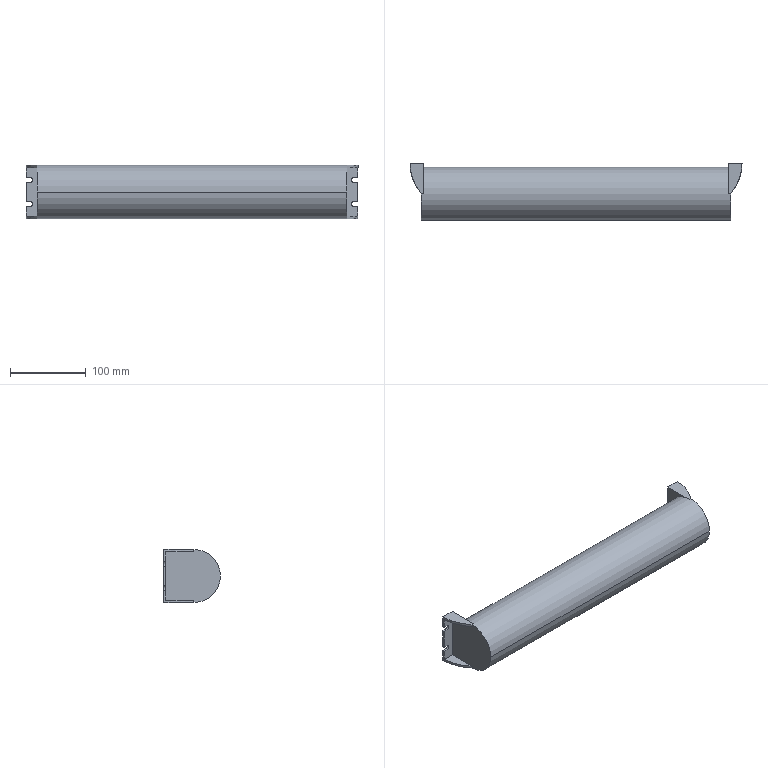Component | SolidWorks | IlluminationLamp-1 | 1 solid | 36 faces | box 438 x 75 x 70 mm | volume 1585479 mm3 | plane 24 | cylinder 12 | commonest cylinder face diameters 121.667 x6 6.5 x4 70 x2
STEP:
#1=COLOUR_RGB('',0.7922,0.8196,0.9333);
#2=FILL_AREA_STYLE_COLOUR('',#1);
#3=FILL_AREA_STYLE('',(#2));
#4=SURFACE_STYLE_FILL_AREA(#3);
#5=SURFACE_SIDE_STYLE('',(#4));
#6=SURFACE_STYLE_USAGE(.BOTH.,#5);
#7=PRESENTATION_STYLE_ASSIGNMENT((#6));
#8=CARTESIAN_POINT('',(8.246,13.054,-8.406));
#9=VERTEX_POINT('',#8);
#10=CARTESIAN_POINT('',(8.246,11.676,-7.028));
#11=VERTEX_POINT('',#10);
#12=CARTESIAN_POINT('',(8.246,13.054,-7.028));
#13=DIRECTION('',(-1.,-0.,0.));
#14=DIRECTION('',(0.,1.,0.));
#15=AXIS2_PLACEMENT_3D('',#12,#13,#14);
#16=CIRCLE('',#15,1.378);
#17=EDGE_CURVE('',#9,#11,#16,.T.);
#18=ORIENTED_EDGE('',*,*,#17,.T.);
#19=CARTESIAN_POINT('',(-7.817,11.676,-7.028));
#20=VERTEX_POINT('',#19);
#21=CARTESIAN_POINT('',(8.246,11.676,-7.028));
#22=DIRECTION('',(-1.,-0.,0.));
#23=VECTOR('',#22,39.37);
#24=LINE('',#21,#23);
#25=EDGE_CURVE('',#11,#20,#24,.T.);
#26=ORIENTED_EDGE('',*,*,#25,.T.);
#27=CARTESIAN_POINT('',(-7.817,13.054,-8.406));
#28=VERTEX_POINT('',#27);
#29=CARTESIAN_POINT('',(-7.817,13.054,-7.028));
#30=DIRECTION('',(1.,0.,-0.));
#31=DIRECTION('',(0.,1.,0.));
#32=AXIS2_PLACEMENT_3D('',#29,#30,#31);
#33=CIRCLE('',#32,1.378);
#34=EDGE_CURVE('',#20,#28,#33,.T.);
#35=ORIENTED_EDGE('',*,*,#34,.T.);
#36=CARTESIAN_POINT('',(-7.699,13.054,-8.406));
#37=VERTEX_POINT('',#36);
#38=CARTESIAN_POINT('',(8.246,13.054,-8.406));
#39=DIRECTION('',(1.,0.,-0.));
#40=VECTOR('',#39,39.37);
#41=LINE('',#38,#40);
#42=EDGE_CURVE('',#28,#37,#41,.T.);
#43=ORIENTED_EDGE('',*,*,#42,.T.);
#44=CARTESIAN_POINT('',(-7.699,14.432,-7.028));
#45=VERTEX_POINT('',#44);
#46=CARTESIAN_POINT('',(-7.699,13.054,-7.028));
#47=DIRECTION('',(1.,0.,-0.));
#48=DIRECTION('',(0.,1.,0.));
#49=AXIS2_PLACEMENT_3D('',#46,#47,#48);
#50=CIRCLE('',#49,1.378);
#51=EDGE_CURVE('',#37,#45,#50,.T.);
#52=ORIENTED_EDGE('',*,*,#51,.T.);
#53=CARTESIAN_POINT('',(8.128,14.432,-7.028));
#54=VERTEX_POINT('',#53);
#55=CARTESIAN_POINT('',(8.246,14.432,-7.028));
#56=DIRECTION('',(-1.,-0.,0.));
#57=VECTOR('',#56,39.37);
#58=LINE('',#55,#57);
#59=EDGE_CURVE('',#54,#45,#58,.T.);
#60=ORIENTED_EDGE('',*,*,#59,.F.);
#61=CARTESIAN_POINT('',(8.128,13.054,-8.406));
#62=VERTEX_POINT('',#61);
#63=CARTESIAN_POINT('',(8.128,13.054,-7.028));
#64=DIRECTION('',(-1.,-0.,0.));
#65=DIRECTION('',(0.,1.,0.));
#66=AXIS2_PLACEMENT_3D('',#63,#64,#65);
#67=CIRCLE('',#66,1.378);
#68=EDGE_CURVE('',#54,#62,#67,.T.);
#69=ORIENTED_EDGE('',*,*,#68,.T.);
#70=CARTESIAN_POINT('',(8.246,13.054,-8.406));
#71=DIRECTION('',(1.,0.,-0.));
#72=VECTOR('',#71,39.37);
#73=LINE('',#70,#72);
#74=EDGE_CURVE('',#62,#9,#73,.T.);
#75=ORIENTED_EDGE('',*,*,#74,.T.);
#76=EDGE_LOOP('',(#18,#26,#35,#43,#52,#60,#69,#75));
#77=FACE_OUTER_BOUND('',#76,.T.);
#78=CARTESIAN_POINT('',(8.246,13.054,-7.028));
#79=DIRECTION('',(-1.,-0.,0.));
#80=DIRECTION('',(0.,1.,0.));
#81=AXIS2_PLACEMENT_3D('',#78,#79,#80);
#82=CYLINDRICAL_SURFACE('',#81,1.378);
#83=ADVANCED_FACE('',(#77),#82,.T.);
#84=ORIENTED_EDGE('',*,*,#25,.F.);
#85=CARTESIAN_POINT('',(8.246,13.054,-5.65));
#86=VERTEX_POINT('',#85);
#87=CARTESIAN_POINT('',(8.246,13.054,-7.028));
#88=DIRECTION('',(-1.,-0.,0.));
#89=DIRECTION('',(0.,1.,0.));
#90=AXIS2_PLACEMENT_3D('',#87,#88,#89);
#91=CIRCLE('',#90,1.378);
#92=EDGE_CURVE('',#11,#86,#91,.T.);
#93=ORIENTED_EDGE('',*,*,#92,.T.);
#94=CARTESIAN_POINT('',(8.128,13.054,-5.65));
#95=VERTEX_POINT('',#94);
#96=CARTESIAN_POINT('',(8.246,13.054,-5.65));
#97=DIRECTION('',(-1.,-0.,0.));
#98=VECTOR('',#97,39.37);
#99=LINE('',#96,#98);
#100=EDGE_CURVE('',#86,#95,#99,.T.);
#101=ORIENTED_EDGE('',*,*,#100,.T.);
#102=CARTESIAN_POINT('',(8.128,13.054,-7.028));
#103=DIRECTION('',(-1.,-0.,0.));
#104=DIRECTION('',(0.,1.,0.));
#105=AXIS2_PLACEMENT_3D('',#102,#103,#104);
#106=CIRCLE('',#105,1.378);
#107=EDGE_CURVE('',#95,#54,#106,.T.);
#108=ORIENTED_EDGE('',*,*,#107,.T.);
#109=ORIENTED_EDGE('',*,*,#59,.T.);
#110=CARTESIAN_POINT('',(-7.699,13.054,-5.65));
#111=VERTEX_POINT('',#110);
#112=CARTESIAN_POINT('',(-7.699,13.054,-7.028));
#113=DIRECTION('',(1.,0.,-0.));
#114=DIRECTION('',(0.,1.,0.));
#115=AXIS2_PLACEMENT_3D('',#112,#113,#114);
#116=CIRCLE('',#115,1.378);
#117=EDGE_CURVE('',#45,#111,#116,.T.);
#118=ORIENTED_EDGE('',*,*,#117,.T.);
#119=CARTESIAN_POINT('',(-7.817,13.054,-5.65));
#120=VERTEX_POINT('',#119);
#121=CARTESIAN_POINT('',(8.246,13.054,-5.65));
#122=DIRECTION('',(-1.,-0.,0.));
#123=VECTOR('',#122,39.37);
#124=LINE('',#121,#123);
#125=EDGE_CURVE('',#111,#120,#124,.T.);
#126=ORIENTED_EDGE('',*,*,#125,.T.);
#127=CARTESIAN_POINT('',(-7.817,13.054,-7.028));
#128=DIRECTION('',(1.,0.,-0.));
#129=DIRECTION('',(0.,1.,0.));
#130=AXIS2_PLACEMENT_3D('',#127,#128,#129);
#131=CIRCLE('',#130,1.378);
#132=EDGE_CURVE('',#120,#20,#131,.T.);
#133=ORIENTED_EDGE('',*,*,#132,.T.);
#134=EDGE_LOOP('',(#84,#93,#101,#108,#109,#118,#126,#133));
#135=FACE_OUTER_BOUND('',#134,.T.);
#136=CARTESIAN_POINT('',(8.246,13.054,-7.028));
#137=DIRECTION('',(-1.,-0.,0.));
#138=DIRECTION('',(0.,1.,0.));
#139=AXIS2_PLACEMENT_3D('',#136,#137,#138);
#140=CYLINDRICAL_SURFACE('',#139,1.378);
#141=ADVANCED_FACE('',(#135),#140,.T.);
#142=CARTESIAN_POINT('',(-7.699,14.629,-8.406));
#143=VERTEX_POINT('',#142);
#144=CARTESIAN_POINT('',(-7.699,13.054,-8.406));
#145=DIRECTION('',(-0.,1.,-0.));
#146=VECTOR('',#145,39.37);
#147=LINE('',#144,#146);
#148=EDGE_CURVE('',#37,#143,#147,.T.);
#149=ORIENTED_EDGE('',*,*,#148,.F.);
#150=ORIENTED_EDGE('',*,*,#42,.F.);
#151=CARTESIAN_POINT('',(-8.407,14.629,-8.406));
#152=VERTEX_POINT('',#151);
#153=CARTESIAN_POINT('',(-6.012,14.629,-8.406));
#154=DIRECTION('',(0.,0.,1.));
#155=DIRECTION('',(0.,1.,0.));
#156=AXIS2_PLACEMENT_3D('',#153,#154,#155);
#157=CIRCLE('',#156,2.395);
#158=EDGE_CURVE('',#152,#28,#157,.T.);
#159=ORIENTED_EDGE('',*,*,#158,.F.);
#160=CARTESIAN_POINT('',(0.2146,14.629,-8.406));
#161=DIRECTION('',(-1.,-0.,0.));
#162=VECTOR('',#161,39.37);
#163=LINE('',#160,#162);
#164=EDGE_CURVE('',#143,#152,#163,.T.);
#165=ORIENTED_EDGE('',*,*,#164,.F.);
#166=EDGE_LOOP('',(#149,#150,#159,#165));
#167=FACE_OUTER_BOUND('',#166,.T.);
#168=CARTESIAN_POINT('',(0.2146,13.054,-8.406));
#169=DIRECTION('',(0.,0.,1.));
#170=DIRECTION('',(-0.,1.,-0.));
#171=AXIS2_PLACEMENT_3D('',#168,#169,#170);
#172=PLANE('',#171);
#173=ADVANCED_FACE('',(#167),#172,.F.);
#174=CARTESIAN_POINT('',(-7.817,14.51,-5.768));
#175=VERTEX_POINT('',#174);
#176=CARTESIAN_POINT('',(-7.817,14.51,-8.288));
#177=VERTEX_POINT('',#176);
#178=CARTESIAN_POINT('',(-7.817,14.51,-7.028));
#179=DIRECTION('',(-0.,-0.,-1.));
#180=VECTOR('',#179,39.37);
#181=LINE('',#178,#180);
#182=EDGE_CURVE('',#175,#177,#181,.T.);
#183=ORIENTED_EDGE('',*,*,#182,.T.);
#184=CARTESIAN_POINT('',(-7.817,13.054,-8.288));
#185=VERTEX_POINT('',#184);
#186=CARTESIAN_POINT('',(-7.817,13.054,-8.288));
#187=DIRECTION('',(0.,-1.,0.));
#188=VECTOR('',#187,39.37);
#189=LINE('',#186,#188);
#190=EDGE_CURVE('',#177,#185,#189,.T.);
#191=ORIENTED_EDGE('',*,*,#190,.T.);
#192=CARTESIAN_POINT('',(-7.817,13.054,-7.028));
#193=DIRECTION('',(-0.,-0.,-1.));
#194=VECTOR('',#193,39.37);
#195=LINE('',#192,#194);
#196=EDGE_CURVE('',#185,#28,#195,.T.);
#197=ORIENTED_EDGE('',*,*,#196,.T.);
#198=ORIENTED_EDGE('',*,*,#34,.F.);
#199=ORIENTED_EDGE('',*,*,#132,.F.);
#200=CARTESIAN_POINT('',(-7.817,13.054,-5.768));
#201=VERTEX_POINT('',#200);
#202=CARTESIAN_POINT('',(-7.817,13.054,-7.028));
#203=DIRECTION('',(-0.,-0.,-1.));
#204=VECTOR('',#203,39.37);
#205=LINE('',#202,#204);
#206=EDGE_CURVE('',#120,#201,#205,.T.);
#207=ORIENTED_EDGE('',*,*,#206,.T.);
#208=CARTESIAN_POINT('',(-7.817,13.054,-5.768));
#209=DIRECTION('',(-0.,1.,-0.));
#210=VECTOR('',#209,39.37);
#211=LINE('',#208,#210);
#212=EDGE_CURVE('',#201,#175,#211,.T.);
#213=ORIENTED_EDGE('',*,*,#212,.T.);
#214=EDGE_LOOP('',(#183,#191,#197,#198,#199,#207,#213));
#215=FACE_OUTER_BOUND('',#214,.T.);
#216=CARTESIAN_POINT('',(-7.817,13.054,-7.028));
#217=DIRECTION('',(-1.,-0.,0.));
#218=DIRECTION('',(-0.,1.,-0.));
#219=AXIS2_PLACEMENT_3D('',#216,#217,#218);
#220=PLANE('',#219);
#221=ADVANCED_FACE('',(#215),#220,.T.);
#222=CARTESIAN_POINT('',(-7.699,14.629,-5.65));
#223=VERTEX_POINT('',#222);
#224=CARTESIAN_POINT('',(-7.699,13.054,-5.65));
#225=DIRECTION('',(-0.,1.,-0.));
#226=VECTOR('',#225,39.37);
#227=LINE('',#224,#226);
#228=EDGE_CURVE('',#111,#223,#227,.T.);
#229=ORIENTED_EDGE('',*,*,#228,.T.);
#230=CARTESIAN_POINT('',(-8.407,14.629,-5.65));
#231=VERTEX_POINT('',#230);
#232=CARTESIAN_POINT('',(0.2146,14.629,-5.65));
#233=DIRECTION('',(-1.,-0.,0.));
#234=VECTOR('',#233,39.37);
#235=LINE('',#232,#234);
#236=EDGE_CURVE('',#223,#231,#235,.T.);
#237=ORIENTED_EDGE('',*,*,#236,.T.);
#238=CARTESIAN_POINT('',(-6.012,14.629,-5.65));
#239=DIRECTION('',(0.,0.,1.));
#240=DIRECTION('',(0.,1.,0.));
#241=AXIS2_PLACEMENT_3D('',#238,#239,#240);
#242=CIRCLE('',#241,2.395);
#243=EDGE_CURVE('',#231,#120,#242,.T.);
#244=ORIENTED_EDGE('',*,*,#243,.T.);
#245=ORIENTED_EDGE('',*,*,#125,.F.);
#246=EDGE_LOOP('',(#229,#237,#244,#245));
#247=FACE_OUTER_BOUND('',#246,.T.);
#248=CARTESIAN_POINT('',(0.2146,13.054,-5.65));
#249=DIRECTION('',(0.,0.,1.));
#250=DIRECTION('',(-0.,1.,-0.));
#251=AXIS2_PLACEMENT_3D('',#248,#249,#250);
#252=PLANE('',#251);
#253=ADVANCED_FACE('',(#247),#252,.T.);
#254=CARTESIAN_POINT('',(8.128,14.629,-5.65));
#255=VERTEX_POINT('',#254);
#256=CARTESIAN_POINT('',(8.128,13.054,-5.65));
#257=DIRECTION('',(-0.,1.,-0.));
#258=VECTOR('',#257,39.37);
#259=LINE('',#256,#258);
#260=EDGE_CURVE('',#95,#255,#259,.T.);
#261=ORIENTED_EDGE('',*,*,#260,.F.);
#262=ORIENTED_EDGE('',*,*,#100,.F.);
#263=CARTESIAN_POINT('',(8.837,14.629,-5.65));
#264=VERTEX_POINT('',#263);
#265=CARTESIAN_POINT('',(6.442,14.629,-5.65));
#266=DIRECTION('',(-0.,-0.,-1.));
#267=DIRECTION('',(0.,-1.,0.));
#268=AXIS2_PLACEMENT_3D('',#265,#266,#267);
#269=CIRCLE('',#268,2.395);
#270=EDGE_CURVE('',#264,#86,#269,.T.);
#271=ORIENTED_EDGE('',*,*,#270,.F.);
#272=CARTESIAN_POINT('',(0.2146,14.629,-5.65));
#273=DIRECTION('',(1.,0.,-0.));
#274=VECTOR('',#273,39.37);
#275=LINE('',#272,#274);
#276=EDGE_CURVE('',#255,#264,#275,.T.);
#277=ORIENTED_EDGE('',*,*,#276,.F.);
#278=EDGE_LOOP('',(#261,#262,#271,#277));
#279=FACE_OUTER_BOUND('',#278,.T.);
#280=CARTESIAN_POINT('',(0.2146,13.054,-5.65));
#281=DIRECTION('',(-0.,-0.,-1.));
#282=DIRECTION('',(0.,-1.,0.));
#283=AXIS2_PLACEMENT_3D('',#280,#281,#282);
#284=PLANE('',#283);
#285=ADVANCED_FACE('',(#279),#284,.F.);
#286=ORIENTED_EDGE('',*,*,#17,.F.);
#287=CARTESIAN_POINT('',(8.246,13.054,-8.288));
#288=VERTEX_POINT('',#287);
#289=CARTESIAN_POINT('',(8.246,13.054,-7.028));
#290=DIRECTION('',(-0.,-0.,-1.));
#291=VECTOR('',#290,39.37);
#292=LINE('',#289,#291);
#293=EDGE_CURVE('',#288,#9,#292,.T.);
#294=ORIENTED_EDGE('',*,*,#293,.F.);
#295=CARTESIAN_POINT('',(8.246,14.51,-8.288));
#296=VERTEX_POINT('',#295);
#297=CARTESIAN_POINT('',(8.246,13.054,-8.288));
#298=DIRECTION('',(0.,-1.,0.));
#299=VECTOR('',#298,39.37);
#300=LINE('',#297,#299);
#301=EDGE_CURVE('',#296,#288,#300,.T.);
#302=ORIENTED_EDGE('',*,*,#301,.F.);
#303=CARTESIAN_POINT('',(8.246,14.51,-5.768));
#304=VERTEX_POINT('',#303);
#305=CARTESIAN_POINT('',(8.246,14.51,-7.028));
#306=DIRECTION('',(-0.,-0.,-1.));
#307=VECTOR('',#306,39.37);
#308=LINE('',#305,#307);
#309=EDGE_CURVE('',#304,#296,#308,.T.);
#310=ORIENTED_EDGE('',*,*,#309,.F.);
#311=CARTESIAN_POINT('',(8.246,13.054,-5.768));
#312=VERTEX_POINT('',#311);
#313=CARTESIAN_POINT('',(8.246,13.054,-5.768));
#314=DIRECTION('',(-0.,1.,-0.));
#315=VECTOR('',#314,39.37);
#316=LINE('',#313,#315);
#317=EDGE_CURVE('',#312,#304,#316,.T.);
#318=ORIENTED_EDGE('',*,*,#317,.F.);
#319=CARTESIAN_POINT('',(8.246,13.054,-7.028));
#320=DIRECTION('',(-0.,-0.,-1.));
#321=VECTOR('',#320,39.37);
#322=LINE('',#319,#321);
#323=EDGE_CURVE('',#86,#312,#322,.T.);
#324=ORIENTED_EDGE('',*,*,#323,.F.);
#325=ORIENTED_EDGE('',*,*,#92,.F.);
#326=EDGE_LOOP('',(#286,#294,#302,#310,#318,#324,#325));
#327=FACE_OUTER_BOUND('',#326,.T.);
#328=CARTESIAN_POINT('',(8.246,13.054,-7.028));
#329=DIRECTION('',(-1.,-0.,0.));
#330=DIRECTION('',(-0.,1.,-0.));
#331=AXIS2_PLACEMENT_3D('',#328,#329,#330);
#332=PLANE('',#331);
#333=ADVANCED_FACE('',(#327),#332,.F.);
#334=CARTESIAN_POINT('',(8.128,14.629,-8.406));
#335=VERTEX_POINT('',#334);
#336=CARTESIAN_POINT('',(8.128,13.054,-8.406));
#337=DIRECTION('',(-0.,1.,-0.));
#338=VECTOR('',#337,39.37);
#339=LINE('',#336,#338);
#340=EDGE_CURVE('',#62,#335,#339,.T.);
#341=ORIENTED_EDGE('',*,*,#340,.T.);
#342=CARTESIAN_POINT('',(8.837,14.629,-8.406));
#343=VERTEX_POINT('',#342);
#344=CARTESIAN_POINT('',(0.2146,14.629,-8.406));
#345=DIRECTION('',(1.,0.,-0.));
#346=VECTOR('',#345,39.37);
#347=LINE('',#344,#346);
#348=EDGE_CURVE('',#335,#343,#347,.T.);
#349=ORIENTED_EDGE('',*,*,#348,.T.);
#350=CARTESIAN_POINT('',(6.442,14.629,-8.406));
#351=DIRECTION('',(-0.,-0.,-1.));
#352=DIRECTION('',(0.,-1.,0.));
#353=AXIS2_PLACEMENT_3D('',#350,#351,#352);
#354=CIRCLE('',#353,2.395);
#355=EDGE_CURVE('',#343,#9,#354,.T.);
#356=ORIENTED_EDGE('',*,*,#355,.T.);
#357=ORIENTED_EDGE('',*,*,#74,.F.);
#358=EDGE_LOOP('',(#341,#349,#356,#357));
#359=FACE_OUTER_BOUND('',#358,.T.);
#360=CARTESIAN_POINT('',(0.2146,13.054,-8.406));
#361=DIRECTION('',(-0.,-0.,-1.));
#362=DIRECTION('',(0.,-1.,0.));
#363=AXIS2_PLACEMENT_3D('',#360,#361,#362);
#364=PLANE('',#363);
#365=ADVANCED_FACE('',(#359),#364,.T.);
#366=ORIENTED_EDGE('',*,*,#236,.F.);
#367=CARTESIAN_POINT('',(-7.699,14.629,-5.65));
#368=DIRECTION('',(0.,0.,1.));
#369=VECTOR('',#368,39.37);
#370=LINE('',#367,#369);
#371=EDGE_CURVE('',#143,#223,#370,.T.);
#372=ORIENTED_EDGE('',*,*,#371,.F.);
#373=ORIENTED_EDGE('',*,*,#164,.T.);
#374=CARTESIAN_POINT('',(-8.407,14.629,-7.786));
#375=VERTEX_POINT('',#374);
#376=CARTESIAN_POINT('',(-8.407,14.629,-5.65));
#377=DIRECTION('',(-0.,-0.,-1.));
#378=VECTOR('',#377,39.37);
#379=LINE('',#376,#378);
#380=EDGE_CURVE('',#375,#152,#379,.T.);
#381=ORIENTED_EDGE('',*,*,#380,.F.);
#382=CARTESIAN_POINT('',(-8.191,14.629,-7.786));
#383=VERTEX_POINT('',#382);
#384=CARTESIAN_POINT('',(-7.817,14.629,-7.786));
#385=DIRECTION('',(-1.,-0.,0.));
#386=VECTOR('',#385,39.37);
#387=LINE('',#384,#386);
#388=EDGE_CURVE('',#383,#375,#387,.T.);
#389=ORIENTED_EDGE('',*,*,#388,.F.);
#390=CARTESIAN_POINT('',(-8.191,14.629,-7.53));
#391=VERTEX_POINT('',#390);
#392=CARTESIAN_POINT('',(-8.191,14.629,-7.658));
#393=DIRECTION('',(-0.,1.,-0.));
#394=DIRECTION('',(0.,0.,-1.));
#395=AXIS2_PLACEMENT_3D('',#392,#393,#394);
#396=CIRCLE('',#395,0.128);
#397=EDGE_CURVE('',#391,#383,#396,.T.);
#398=ORIENTED_EDGE('',*,*,#397,.F.);
#399=CARTESIAN_POINT('',(-8.407,14.629,-7.53));
#400=VERTEX_POINT('',#399);
#401=CARTESIAN_POINT('',(-7.817,14.629,-7.53));
#402=DIRECTION('',(1.,0.,-0.));
#403=VECTOR('',#402,39.37);
#404=LINE('',#401,#403);
#405=EDGE_CURVE('',#400,#391,#404,.T.);
#406=ORIENTED_EDGE('',*,*,#405,.F.);
#407=CARTESIAN_POINT('',(-8.407,14.629,-6.526));
#408=VERTEX_POINT('',#407);
#409=CARTESIAN_POINT('',(-8.407,14.629,-5.65));
#410=DIRECTION('',(-0.,-0.,-1.));
#411=VECTOR('',#410,39.37);
#412=LINE('',#409,#411);
#413=EDGE_CURVE('',#408,#400,#412,.T.);
#414=ORIENTED_EDGE('',*,*,#413,.F.);
#415=CARTESIAN_POINT('',(-8.191,14.629,-6.526));
#416=VERTEX_POINT('',#415);
#417=CARTESIAN_POINT('',(-7.817,14.629,-6.526));
#418=DIRECTION('',(-1.,-0.,0.));
#419=VECTOR('',#418,39.37);
#420=LINE('',#417,#419);
#421=EDGE_CURVE('',#416,#408,#420,.T.);
#422=ORIENTED_EDGE('',*,*,#421,.F.);
#423=CARTESIAN_POINT('',(-8.191,14.629,-6.27));
#424=VERTEX_POINT('',#423);
#425=CARTESIAN_POINT('',(-8.191,14.629,-6.398));
#426=DIRECTION('',(-0.,1.,-0.));
#427=DIRECTION('',(0.,0.,-1.));
#428=AXIS2_PLACEMENT_3D('',#425,#426,#427);
#429=CIRCLE('',#428,0.128);
#430=EDGE_CURVE('',#424,#416,#429,.T.);
#431=ORIENTED_EDGE('',*,*,#430,.F.);
#432=CARTESIAN_POINT('',(-8.407,14.629,-6.27));
#433=VERTEX_POINT('',#432);
#434=CARTESIAN_POINT('',(-7.817,14.629,-6.27));
#435=DIRECTION('',(1.,0.,-0.));
#436=VECTOR('',#435,39.37);
#437=LINE('',#434,#436);
#438=EDGE_CURVE('',#433,#424,#437,.T.);
#439=ORIENTED_EDGE('',*,*,#438,.F.);
#440=CARTESIAN_POINT('',(-8.407,14.629,-5.65));
#441=DIRECTION('',(-0.,-0.,-1.));
#442=VECTOR('',#441,39.37);
#443=LINE('',#440,#442);
#444=EDGE_CURVE('',#231,#433,#443,.T.);
#445=ORIENTED_EDGE('',*,*,#444,.F.);
#446=EDGE_LOOP('',(#366,#372,#373,#381,#389,#398,#406,#414,#422,#431,#439,#445));
#447=FACE_OUTER_BOUND('',#446,.T.);
#448=CARTESIAN_POINT('',(-7.817,14.629,-5.65));
#449=DIRECTION('',(0.,-1.,0.));
#450=DIRECTION('',(0.,0.,1.));
#451=AXIS2_PLACEMENT_3D('',#448,#449,#450);
#452=PLANE('',#451);
#453=ADVANCED_FACE('',(#447),#452,.F.);
#454=ORIENTED_EDGE('',*,*,#51,.F.);
#455=ORIENTED_EDGE('',*,*,#148,.T.);
#456=ORIENTED_EDGE('',*,*,#371,.T.);
#457=ORIENTED_EDGE('',*,*,#228,.F.);
#458=ORIENTED_EDGE('',*,*,#117,.F.);
#459=EDGE_LOOP('',(#454,#455,#456,#457,#458));
#460=FACE_OUTER_BOUND('',#459,.T.);
#461=CARTESIAN_POINT('',(-7.699,13.054,-7.028));
#462=DIRECTION('',(1.,0.,-0.));
#463=DIRECTION('',(0.,-1.,0.));
#464=AXIS2_PLACEMENT_3D('',#461,#462,#463);
#465=PLANE('',#464);
#466=ADVANCED_FACE('',(#460),#465,.T.);
#467=CARTESIAN_POINT('',(-8.405,14.51,-8.288));
#468=VERTEX_POINT('',#467);
#469=CARTESIAN_POINT('',(-8.405,14.51,-7.786));
#470=VERTEX_POINT('',#469);
#471=CARTESIAN_POINT('',(-8.405,14.51,-5.65));
#472=DIRECTION('',(0.,0.,1.));
#473=VECTOR('',#472,39.37);
#474=LINE('',#471,#473);
#475=EDGE_CURVE('',#468,#470,#474,.T.);
#476=ORIENTED_EDGE('',*,*,#475,.T.);
#477=CARTESIAN_POINT('',(-6.012,14.629,-7.786));
#478=DIRECTION('',(-0.,-0.,-1.));
#479=DIRECTION('',(-0.,1.,0.));
#480=AXIS2_PLACEMENT_3D('',#477,#478,#479);
#481=CIRCLE('',#480,2.395);
#482=EDGE_CURVE('',#470,#375,#481,.T.);
#483=ORIENTED_EDGE('',*,*,#482,.T.);
#484=ORIENTED_EDGE('',*,*,#380,.T.);
#485=ORIENTED_EDGE('',*,*,#158,.T.);
#486=ORIENTED_EDGE('',*,*,#196,.F.);
#487=CARTESIAN_POINT('',(-6.012,14.629,-8.288));
#488=DIRECTION('',(-0.,-0.,-1.));
#489=DIRECTION('',(0.,1.,0.));
#490=AXIS2_PLACEMENT_3D('',#487,#488,#489);
#491=CIRCLE('',#490,2.395);
#492=EDGE_CURVE('',#185,#468,#491,.T.);
#493=ORIENTED_EDGE('',*,*,#492,.T.);
#494=EDGE_LOOP('',(#476,#483,#484,#485,#486,#493));
#495=FACE_OUTER_BOUND('',#494,.T.);
#496=CARTESIAN_POINT('',(-6.012,14.629,-5.65));
#497=DIRECTION('',(0.,0.,1.));
#498=DIRECTION('',(0.,1.,0.));
#499=AXIS2_PLACEMENT_3D('',#496,#497,#498);
#500=CYLINDRICAL_SURFACE('',#499,2.395);
#501=ADVANCED_FACE('',(#495),#500,.T.);
#502=ORIENTED_EDGE('',*,*,#492,.F.);
#503=ORIENTED_EDGE('',*,*,#190,.F.);
#504=CARTESIAN_POINT('',(0.2146,14.51,-8.288));
#505=DIRECTION('',(-1.,-0.,0.));
#506=VECTOR('',#505,39.37);
#507=LINE('',#504,#506);
#508=EDGE_CURVE('',#177,#468,#507,.T.);
#509=ORIENTED_EDGE('',*,*,#508,.T.);
#510=EDGE_LOOP('',(#502,#503,#509));
#511=FACE_OUTER_BOUND('',#510,.T.);
#512=CARTESIAN_POINT('',(0.2146,13.054,-8.288));
#513=DIRECTION('',(0.,0.,1.));
#514=DIRECTION('',(-0.,1.,-0.));
#515=AXIS2_PLACEMENT_3D('',#512,#513,#514);
#516=PLANE('',#515);
#517=ADVANCED_FACE('',(#511),#516,.T.);
#518=CARTESIAN_POINT('',(-8.405,14.51,-5.768));
#519=VERTEX_POINT('',#518);
#520=CARTESIAN_POINT('',(-8.405,14.51,-6.27));
#521=VERTEX_POINT('',#520);
#522=CARTESIAN_POINT('',(-8.405,14.51,-5.768));
#523=DIRECTION('',(-0.,-0.,-1.));
#524=VECTOR('',#523,39.37);
#525=LINE('',#522,#524);
#526=EDGE_CURVE('',#519,#521,#525,.T.);
#527=ORIENTED_EDGE('',*,*,#526,.T.);
#528=CARTESIAN_POINT('',(-8.191,14.51,-6.27));
#529=VERTEX_POINT('',#528);
#530=CARTESIAN_POINT('',(-7.817,14.51,-6.27));
#531=DIRECTION('',(1.,0.,-0.));
#532=VECTOR('',#531,39.37);
#533=LINE('',#530,#532);
#534=EDGE_CURVE('',#521,#529,#533,.T.);
#535=ORIENTED_EDGE('',*,*,#534,.T.);
#536=CARTESIAN_POINT('',(-8.191,14.51,-6.526));
#537=VERTEX_POINT('',#536);
#538=CARTESIAN_POINT('',(-8.191,14.51,-6.398));
#539=DIRECTION('',(-0.,1.,-0.));
#540=DIRECTION('',(0.,0.,-1.));
#541=AXIS2_PLACEMENT_3D('',#538,#539,#540);
#542=CIRCLE('',#541,0.128);
#543=EDGE_CURVE('',#529,#537,#542,.T.);
#544=ORIENTED_EDGE('',*,*,#543,.T.);
#545=CARTESIAN_POINT('',(-8.405,14.51,-6.526));
#546=VERTEX_POINT('',#545);
#547=CARTESIAN_POINT('',(-7.817,14.51,-6.526));
#548=DIRECTION('',(-1.,-0.,0.));
#549=VECTOR('',#548,39.37);
#550=LINE('',#547,#549);
#551=EDGE_CURVE('',#537,#546,#550,.T.);
#552=ORIENTED_EDGE('',*,*,#551,.T.);
#553=CARTESIAN_POINT('',(-8.405,14.51,-7.53));
#554=VERTEX_POINT('',#553);
#555=CARTESIAN_POINT('',(-8.405,14.51,-5.768));
#556=DIRECTION('',(-0.,-0.,-1.));
#557=VECTOR('',#556,39.37);
#558=LINE('',#555,#557);
#559=EDGE_CURVE('',#546,#554,#558,.T.);
#560=ORIENTED_EDGE('',*,*,#559,.T.);
#561=CARTESIAN_POINT('',(-8.191,14.51,-7.53));
#562=VERTEX_POINT('',#561);
#563=CARTESIAN_POINT('',(-7.817,14.51,-7.53));
#564=DIRECTION('',(1.,0.,-0.));
#565=VECTOR('',#564,39.37);
#566=LINE('',#563,#565);
#567=EDGE_CURVE('',#554,#562,#566,.T.);
#568=ORIENTED_EDGE('',*,*,#567,.T.);
#569=CARTESIAN_POINT('',(-8.191,14.51,-7.786));
#570=VERTEX_POINT('',#569);
#571=CARTESIAN_POINT('',(-8.191,14.51,-7.658));
#572=DIRECTION('',(-0.,1.,-0.));
#573=DIRECTION('',(0.,0.,-1.));
#574=AXIS2_PLACEMENT_3D('',#571,#572,#573);
#575=CIRCLE('',#574,0.128);
#576=EDGE_CURVE('',#562,#570,#575,.T.);
#577=ORIENTED_EDGE('',*,*,#576,.T.);
#578=CARTESIAN_POINT('',(-7.817,14.51,-7.786));
#579=DIRECTION('',(-1.,-0.,0.));
#580=VECTOR('',#579,39.37);
#581=LINE('',#578,#580);
#582=EDGE_CURVE('',#570,#470,#581,.T.);
#583=ORIENTED_EDGE('',*,*,#582,.T.);
#584=ORIENTED_EDGE('',*,*,#475,.F.);
#585=ORIENTED_EDGE('',*,*,#508,.F.);
#586=ORIENTED_EDGE('',*,*,#182,.F.);
#587=CARTESIAN_POINT('',(-7.817,14.51,-5.768));
#588=DIRECTION('',(-1.,-0.,0.));
#589=VECTOR('',#588,39.37);
#590=LINE('',#587,#589);
#591=EDGE_CURVE('',#175,#519,#590,.T.);
#592=ORIENTED_EDGE('',*,*,#591,.T.);
#593=EDGE_LOOP('',(#527,#535,#544,#552,#560,#568,#577,#583,#584,#585,#586,#592));
#594=FACE_OUTER_BOUND('',#593,.T.);
#595=CARTESIAN_POINT('',(-7.817,14.51,-5.768));
#596=DIRECTION('',(0.,-1.,0.));
#597=DIRECTION('',(0.,0.,1.));
#598=AXIS2_PLACEMENT_3D('',#595,#596,#597);
#599=PLANE('',#598);
#600=ADVANCED_FACE('',(#594),#599,.T.);
#601=ORIENTED_EDGE('',*,*,#591,.F.);
#602=ORIENTED_EDGE('',*,*,#212,.F.);
#603=CARTESIAN_POINT('',(-6.012,14.629,-5.768));
#604=DIRECTION('',(0.,0.,1.));
#605=DIRECTION('',(0.,1.,0.));
#606=AXIS2_PLACEMENT_3D('',#603,#604,#605);
#607=CIRCLE('',#606,2.395);
#608=EDGE_CURVE('',#519,#201,#607,.T.);
#609=ORIENTED_EDGE('',*,*,#608,.F.);
#610=EDGE_LOOP('',(#601,#602,#609));
#611=FACE_OUTER_BOUND('',#610,.T.);
#612=CARTESIAN_POINT('',(0.2146,13.054,-5.768));
#613=DIRECTION('',(0.,0.,1.));
#614=DIRECTION('',(-0.,1.,-0.));
#615=AXIS2_PLACEMENT_3D('',#612,#613,#614);
#616=PLANE('',#615);
#617=ADVANCED_FACE('',(#611),#616,.F.);
#618=ORIENTED_EDGE('',*,*,#444,.T.);
#619=CARTESIAN_POINT('',(-6.012,14.629,-6.27));
#620=DIRECTION('',(0.,0.,1.));
#621=DIRECTION('',(0.,1.,0.));
#622=AXIS2_PLACEMENT_3D('',#619,#620,#621);
#623=CIRCLE('',#622,2.395);
#624=EDGE_CURVE('',#433,#521,#623,.T.);
#625=ORIENTED_EDGE('',*,*,#624,.T.);
#626=ORIENTED_EDGE('',*,*,#526,.F.);
#627=ORIENTED_EDGE('',*,*,#608,.T.);
#628=ORIENTED_EDGE('',*,*,#206,.F.);
#629=ORIENTED_EDGE('',*,*,#243,.F.);
#630=EDGE_LOOP('',(#618,#625,#626,#627,#628,#629));
#631=FACE_OUTER_BOUND('',#630,.T.);
#632=CARTESIAN_POINT('',(-6.012,14.629,-5.65));
#633=DIRECTION('',(0.,0.,1.));
#634=DIRECTION('',(0.,1.,0.));
#635=AXIS2_PLACEMENT_3D('',#632,#633,#634);
#636=CYLINDRICAL_SURFACE('',#635,2.395);
#637=ADVANCED_FACE('',(#631),#636,.T.);
#638=CARTESIAN_POINT('',(8.128,14.629,-7.028));
#639=DIRECTION('',(0.,0.,1.));
#640=VECTOR('',#639,39.37);
#641=LINE('',#638,#640);
#642=EDGE_CURVE('',#335,#255,#641,.T.);
#643=ORIENTED_EDGE('',*,*,#642,.F.);
#644=ORIENTED_EDGE('',*,*,#340,.F.);
#645=ORIENTED_EDGE('',*,*,#68,.F.);
#646=ORIENTED_EDGE('',*,*,#107,.F.);
#647=ORIENTED_EDGE('',*,*,#260,.T.);
#648=EDGE_LOOP('',(#643,#644,#645,#646,#647));
#649=FACE_OUTER_BOUND('',#648,.T.);
#650=CARTESIAN_POINT('',(8.128,13.054,-7.028));
#651=DIRECTION('',(1.,0.,-0.));
#652=DIRECTION('',(0.,-1.,0.));
#653=AXIS2_PLACEMENT_3D('',#650,#651,#652);
#654=PLANE('',#653);
#655=ADVANCED_FACE('',(#649),#654,.F.);
#656=CARTESIAN_POINT('',(8.837,14.629,-6.27));
#657=VERTEX_POINT('',#656);
#658=CARTESIAN_POINT('',(8.837,14.629,-5.65));
#659=DIRECTION('',(-0.,-0.,-1.));
#660=VECTOR('',#659,39.37);
#661=LINE('',#658,#660);
#662=EDGE_CURVE('',#264,#657,#661,.T.);
#663=ORIENTED_EDGE('',*,*,#662,.T.);
#664=CARTESIAN_POINT('',(8.62,14.629,-6.27));
#665=VERTEX_POINT('',#664);
#666=CARTESIAN_POINT('',(8.246,14.629,-6.27));
#667=DIRECTION('',(-1.,-0.,0.));
#668=VECTOR('',#667,39.37);
#669=LINE('',#666,#668);
#670=EDGE_CURVE('',#657,#665,#669,.T.);
#671=ORIENTED_EDGE('',*,*,#670,.T.);
#672=CARTESIAN_POINT('',(8.62,14.629,-6.526));
#673=VERTEX_POINT('',#672);
#674=CARTESIAN_POINT('',(8.62,14.629,-6.398));
#675=DIRECTION('',(0.,-1.,0.));
#676=DIRECTION('',(0.,0.,1.));
#677=AXIS2_PLACEMENT_3D('',#674,#675,#676);
#678=CIRCLE('',#677,0.128);
#679=EDGE_CURVE('',#665,#673,#678,.T.);
#680=ORIENTED_EDGE('',*,*,#679,.T.);
#681=CARTESIAN_POINT('',(8.837,14.629,-6.526));
#682=VERTEX_POINT('',#681);
#683=CARTESIAN_POINT('',(8.246,14.629,-6.526));
#684=DIRECTION('',(1.,0.,-0.));
#685=VECTOR('',#684,39.37);
#686=LINE('',#683,#685);
#687=EDGE_CURVE('',#673,#682,#686,.T.);
#688=ORIENTED_EDGE('',*,*,#687,.T.);
#689=CARTESIAN_POINT('',(8.837,14.629,-7.53));
#690=VERTEX_POINT('',#689);
#691=CARTESIAN_POINT('',(8.837,14.629,-5.65));
#692=DIRECTION('',(-0.,-0.,-1.));
#693=VECTOR('',#692,39.37);
#694=LINE('',#691,#693);
#695=EDGE_CURVE('',#682,#690,#694,.T.);
#696=ORIENTED_EDGE('',*,*,#695,.T.);
#697=CARTESIAN_POINT('',(8.62,14.629,-7.53));
#698=VERTEX_POINT('',#697);
#699=CARTESIAN_POINT('',(8.246,14.629,-7.53));
#700=DIRECTION('',(-1.,-0.,0.));
#701=VECTOR('',#700,39.37);
#702=LINE('',#699,#701);
#703=EDGE_CURVE('',#690,#698,#702,.T.);
#704=ORIENTED_EDGE('',*,*,#703,.T.);
#705=CARTESIAN_POINT('',(8.62,14.629,-7.786));
#706=VERTEX_POINT('',#705);
#707=CARTESIAN_POINT('',(8.62,14.629,-7.658));
#708=DIRECTION('',(0.,-1.,0.));
#709=DIRECTION('',(0.,0.,1.));
#710=AXIS2_PLACEMENT_3D('',#707,#708,#709);
#711=CIRCLE('',#710,0.128);
#712=EDGE_CURVE('',#698,#706,#711,.T.);
#713=ORIENTED_EDGE('',*,*,#712,.T.);
#714=CARTESIAN_POINT('',(8.837,14.629,-7.786));
#715=VERTEX_POINT('',#714);
#716=CARTESIAN_POINT('',(8.246,14.629,-7.786));
#717=DIRECTION('',(1.,0.,-0.));
#718=VECTOR('',#717,39.37);
#719=LINE('',#716,#718);
#720=EDGE_CURVE('',#706,#715,#719,.T.);
#721=ORIENTED_EDGE('',*,*,#720,.T.);
#722=CARTESIAN_POINT('',(8.837,14.629,-5.65));
#723=DIRECTION('',(-0.,-0.,-1.));
#724=VECTOR('',#723,39.37);
#725=LINE('',#722,#724);
#726=EDGE_CURVE('',#715,#343,#725,.T.);
#727=ORIENTED_EDGE('',*,*,#726,.T.);
#728=ORIENTED_EDGE('',*,*,#348,.F.);
#729=ORIENTED_EDGE('',*,*,#642,.T.);
#730=ORIENTED_EDGE('',*,*,#276,.T.);
#731=EDGE_LOOP('',(#663,#671,#680,#688,#696,#704,#713,#721,#727,#728,#729,#730));
#732=FACE_OUTER_BOUND('',#731,.T.);
#733=CARTESIAN_POINT('',(8.246,14.629,-5.65));
#734=DIRECTION('',(-0.,1.,-0.));
#735=DIRECTION('',(-0.,-0.,-1.));
#736=AXIS2_PLACEMENT_3D('',#733,#734,#735);
#737=PLANE('',#736);
#738=ADVANCED_FACE('',(#732),#737,.T.);
#739=CARTESIAN_POINT('',(8.834,14.51,-5.768));
#740=VERTEX_POINT('',#739);
#741=CARTESIAN_POINT('',(6.442,14.629,-5.768));
#742=DIRECTION('',(0.,0.,1.));
#743=DIRECTION('',(0.,-1.,0.));
#744=AXIS2_PLACEMENT_3D('',#741,#742,#743);
#745=CIRCLE('',#744,2.395);
#746=EDGE_CURVE('',#312,#740,#745,.T.);
#747=ORIENTED_EDGE('',*,*,#746,.T.);
#748=CARTESIAN_POINT('',(8.834,14.51,-6.27));
#749=VERTEX_POINT('',#748);
#750=CARTESIAN_POINT('',(8.834,14.51,-5.65));
#751=DIRECTION('',(-0.,-0.,-1.));
#752=VECTOR('',#751,39.37);
#753=LINE('',#750,#752);
#754=EDGE_CURVE('',#740,#749,#753,.T.);
#755=ORIENTED_EDGE('',*,*,#754,.T.);
#756=CARTESIAN_POINT('',(6.442,14.629,-6.27));
#757=DIRECTION('',(0.,0.,1.));
#758=DIRECTION('',(-0.,-1.,0.));
#759=AXIS2_PLACEMENT_3D('',#756,#757,#758);
#760=CIRCLE('',#759,2.395);
#761=EDGE_CURVE('',#749,#657,#760,.T.);
#762=ORIENTED_EDGE('',*,*,#761,.T.);
#763=ORIENTED_EDGE('',*,*,#662,.F.);
#764=ORIENTED_EDGE('',*,*,#270,.T.);
#765=ORIENTED_EDGE('',*,*,#323,.T.);
#766=EDGE_LOOP('',(#747,#755,#762,#763,#764,#765));
#767=FACE_OUTER_BOUND('',#766,.T.);
#768=CARTESIAN_POINT('',(6.442,14.629,-5.65));
#769=DIRECTION('',(-0.,-0.,-1.));
#770=DIRECTION('',(0.,-1.,0.));
#771=AXIS2_PLACEMENT_3D('',#768,#769,#770);
#772=CYLINDRICAL_SURFACE('',#771,2.395);
#773=ADVANCED_FACE('',(#767),#772,.T.);
#774=CARTESIAN_POINT('',(8.834,14.51,-7.786));
#775=VERTEX_POINT('',#774);
#776=CARTESIAN_POINT('',(6.442,14.629,-7.786));
#777=DIRECTION('',(-0.,-0.,-1.));
#778=DIRECTION('',(0.,-1.,0.));
#779=AXIS2_PLACEMENT_3D('',#776,#777,#778);
#780=CIRCLE('',#779,2.395);
#781=EDGE_CURVE('',#715,#775,#780,.T.);
#782=ORIENTED_EDGE('',*,*,#781,.T.);
#783=CARTESIAN_POINT('',(8.834,14.51,-8.288));
#784=VERTEX_POINT('',#783);
#785=CARTESIAN_POINT('',(8.834,14.51,-5.65));
#786=DIRECTION('',(-0.,-0.,-1.));
#787=VECTOR('',#786,39.37);
#788=LINE('',#785,#787);
#789=EDGE_CURVE('',#775,#784,#788,.T.);
#790=ORIENTED_EDGE('',*,*,#789,.T.);
#791=CARTESIAN_POINT('',(6.442,14.629,-8.288));
#792=DIRECTION('',(-0.,-0.,-1.));
#793=DIRECTION('',(0.,-1.,0.));
#794=AXIS2_PLACEMENT_3D('',#791,#792,#793);
#795=CIRCLE('',#794,2.395);
#796=EDGE_CURVE('',#784,#288,#795,.T.);
#797=ORIENTED_EDGE('',*,*,#796,.T.);
#798=ORIENTED_EDGE('',*,*,#293,.T.);
#799=ORIENTED_EDGE('',*,*,#355,.F.);
#800=ORIENTED_EDGE('',*,*,#726,.F.);
#801=EDGE_LOOP('',(#782,#790,#797,#798,#799,#800));
#802=FACE_OUTER_BOUND('',#801,.T.);
#803=CARTESIAN_POINT('',(6.442,14.629,-5.65));
#804=DIRECTION('',(-0.,-0.,-1.));
#805=DIRECTION('',(0.,-1.,0.));
#806=AXIS2_PLACEMENT_3D('',#803,#804,#805);
#807=CYLINDRICAL_SURFACE('',#806,2.395);
#808=ADVANCED_FACE('',(#802),#807,.T.);
#809=CARTESIAN_POINT('',(0.2146,14.51,-8.288));
#810=DIRECTION('',(1.,0.,-0.));
#811=VECTOR('',#810,39.37);
#812=LINE('',#809,#811);
#813=EDGE_CURVE('',#296,#784,#812,.T.);
#814=ORIENTED_EDGE('',*,*,#813,.F.);
#815=ORIENTED_EDGE('',*,*,#301,.T.);
#816=ORIENTED_EDGE('',*,*,#796,.F.);
#817=EDGE_LOOP('',(#814,#815,#816));
#818=FACE_OUTER_BOUND('',#817,.T.);
#819=CARTESIAN_POINT('',(0.2146,13.054,-8.288));
#820=DIRECTION('',(-0.,-0.,-1.));
#821=DIRECTION('',(0.,-1.,0.));
#822=AXIS2_PLACEMENT_3D('',#819,#820,#821);
#823=PLANE('',#822);
#824=ADVANCED_FACE('',(#818),#823,.F.);
#825=CARTESIAN_POINT('',(8.246,14.51,-5.768));
#826=DIRECTION('',(1.,0.,-0.));
#827=VECTOR('',#826,39.37);
#828=LINE('',#825,#827);
#829=EDGE_CURVE('',#304,#740,#828,.T.);
#830=ORIENTED_EDGE('',*,*,#829,.F.);
#831=ORIENTED_EDGE('',*,*,#309,.T.);
#832=ORIENTED_EDGE('',*,*,#813,.T.);
#833=ORIENTED_EDGE('',*,*,#789,.F.);
#834=CARTESIAN_POINT('',(8.62,14.51,-7.786));
#835=VERTEX_POINT('',#834);
#836=CARTESIAN_POINT('',(8.246,14.51,-7.786));
#837=DIRECTION('',(1.,0.,-0.));
#838=VECTOR('',#837,39.37);
#839=LINE('',#836,#838);
#840=EDGE_CURVE('',#835,#775,#839,.T.);
#841=ORIENTED_EDGE('',*,*,#840,.F.);
#842=CARTESIAN_POINT('',(8.62,14.51,-7.53));
#843=VERTEX_POINT('',#842);
#844=CARTESIAN_POINT('',(8.62,14.51,-7.658));
#845=DIRECTION('',(0.,-1.,0.));
#846=DIRECTION('',(0.,0.,1.));
#847=AXIS2_PLACEMENT_3D('',#844,#845,#846);
#848=CIRCLE('',#847,0.128);
#849=EDGE_CURVE('',#843,#835,#848,.T.);
#850=ORIENTED_EDGE('',*,*,#849,.F.);
#851=CARTESIAN_POINT('',(8.834,14.51,-7.53));
#852=VERTEX_POINT('',#851);
#853=CARTESIAN_POINT('',(8.246,14.51,-7.53));
#854=DIRECTION('',(-1.,-0.,0.));
#855=VECTOR('',#854,39.37);
#856=LINE('',#853,#855);
#857=EDGE_CURVE('',#852,#843,#856,.T.);
#858=ORIENTED_EDGE('',*,*,#857,.F.);
#859=CARTESIAN_POINT('',(8.834,14.51,-6.526));
#860=VERTEX_POINT('',#859);
#861=CARTESIAN_POINT('',(8.834,14.51,-5.768));
#862=DIRECTION('',(-0.,-0.,-1.));
#863=VECTOR('',#862,39.37);
#864=LINE('',#861,#863);
#865=EDGE_CURVE('',#860,#852,#864,.T.);
#866=ORIENTED_EDGE('',*,*,#865,.F.);
#867=CARTESIAN_POINT('',(8.62,14.51,-6.526));
#868=VERTEX_POINT('',#867);
#869=CARTESIAN_POINT('',(8.246,14.51,-6.526));
#870=DIRECTION('',(1.,0.,-0.));
#871=VECTOR('',#870,39.37);
#872=LINE('',#869,#871);
#873=EDGE_CURVE('',#868,#860,#872,.T.);
#874=ORIENTED_EDGE('',*,*,#873,.F.);
#875=CARTESIAN_POINT('',(8.62,14.51,-6.27));
#876=VERTEX_POINT('',#875);
#877=CARTESIAN_POINT('',(8.62,14.51,-6.398));
#878=DIRECTION('',(0.,-1.,0.));
#879=DIRECTION('',(0.,0.,1.));
#880=AXIS2_PLACEMENT_3D('',#877,#878,#879);
#881=CIRCLE('',#880,0.128);
#882=EDGE_CURVE('',#876,#868,#881,.T.);
#883=ORIENTED_EDGE('',*,*,#882,.F.);
#884=CARTESIAN_POINT('',(8.246,14.51,-6.27));
#885=DIRECTION('',(-1.,-0.,0.));
#886=VECTOR('',#885,39.37);
#887=LINE('',#884,#886);
#888=EDGE_CURVE('',#749,#876,#887,.T.);
#889=ORIENTED_EDGE('',*,*,#888,.F.);
#890=ORIENTED_EDGE('',*,*,#754,.F.);
#891=EDGE_LOOP('',(#830,#831,#832,#833,#841,#850,#858,#866,#874,#883,#889,#890));
#892=FACE_OUTER_BOUND('',#891,.T.);
#893=CARTESIAN_POINT('',(8.246,14.51,-5.768));
#894=DIRECTION('',(-0.,1.,-0.));
#895=DIRECTION('',(-0.,-0.,-1.));
#896=AXIS2_PLACEMENT_3D('',#893,#894,#895);
#897=PLANE('',#896);
#898=ADVANCED_FACE('',(#892),#897,.F.);
#899=ORIENTED_EDGE('',*,*,#746,.F.);
#900=ORIENTED_EDGE('',*,*,#317,.T.);
#901=ORIENTED_EDGE('',*,*,#829,.T.);
#902=EDGE_LOOP('',(#899,#900,#901));
#903=FACE_OUTER_BOUND('',#902,.T.);
#904=CARTESIAN_POINT('',(0.2146,13.054,-5.768));
#905=DIRECTION('',(-0.,-0.,-1.));
#906=DIRECTION('',(0.,-1.,0.));
#907=AXIS2_PLACEMENT_3D('',#904,#905,#906);
#908=PLANE('',#907);
#909=ADVANCED_FACE('',(#903),#908,.T.);
#910=ORIENTED_EDGE('',*,*,#582,.F.);
#911=CARTESIAN_POINT('',(-8.191,14.51,-7.786));
#912=DIRECTION('',(-0.,1.,-0.));
#913=VECTOR('',#912,39.37);
#914=LINE('',#911,#913);
#915=EDGE_CURVE('',#570,#383,#914,.T.);
#916=ORIENTED_EDGE('',*,*,#915,.T.);
#917=ORIENTED_EDGE('',*,*,#388,.T.);
#918=ORIENTED_EDGE('',*,*,#482,.F.);
#919=EDGE_LOOP('',(#910,#916,#917,#918));
#920=FACE_OUTER_BOUND('',#919,.T.);
#921=CARTESIAN_POINT('',(-8.191,14.51,-7.786));
#922=DIRECTION('',(0.,0.,1.));
#923=DIRECTION('',(-0.,1.,-0.));
#924=AXIS2_PLACEMENT_3D('',#921,#922,#923);
#925=PLANE('',#924);
#926=ADVANCED_FACE('',(#920),#925,.T.);
#927=ORIENTED_EDGE('',*,*,#915,.F.);
#928=ORIENTED_EDGE('',*,*,#576,.F.);
#929=CARTESIAN_POINT('',(-8.191,14.51,-7.53));
#930=DIRECTION('',(0.,-1.,0.));
#931=VECTOR('',#930,39.37);
#932=LINE('',#929,#931);
#933=EDGE_CURVE('',#391,#562,#932,.T.);
#934=ORIENTED_EDGE('',*,*,#933,.F.);
#935=ORIENTED_EDGE('',*,*,#397,.T.);
#936=EDGE_LOOP('',(#927,#928,#934,#935));
#937=FACE_OUTER_BOUND('',#936,.T.);
#938=CARTESIAN_POINT('',(-8.191,14.51,-7.658));
#939=DIRECTION('',(-0.,1.,-0.));
#940=DIRECTION('',(0.,0.,-1.));
#941=AXIS2_PLACEMENT_3D('',#938,#939,#940);
#942=CYLINDRICAL_SURFACE('',#941,0.128);
#943=ADVANCED_FACE('',(#937),#942,.F.);
#944=ORIENTED_EDGE('',*,*,#405,.T.);
#945=ORIENTED_EDGE('',*,*,#933,.T.);
#946=ORIENTED_EDGE('',*,*,#567,.F.);
#947=CARTESIAN_POINT('',(-6.012,14.629,-7.53));
#948=DIRECTION('',(-0.,-0.,-1.));
#949=DIRECTION('',(-0.,1.,0.));
#950=AXIS2_PLACEMENT_3D('',#947,#948,#949);
#951=CIRCLE('',#950,2.395);
#952=EDGE_CURVE('',#554,#400,#951,.T.);
#953=ORIENTED_EDGE('',*,*,#952,.T.);
#954=EDGE_LOOP('',(#944,#945,#946,#953));
#955=FACE_OUTER_BOUND('',#954,.T.);
#956=CARTESIAN_POINT('',(-8.588,14.51,-7.53));
#957=DIRECTION('',(-0.,-0.,-1.));
#958=DIRECTION('',(0.,-1.,0.));
#959=AXIS2_PLACEMENT_3D('',#956,#957,#958);
#960=PLANE('',#959);
#961=ADVANCED_FACE('',(#955),#960,.T.);
#962=ORIENTED_EDGE('',*,*,#559,.F.);
#963=CARTESIAN_POINT('',(-6.012,14.629,-6.526));
#964=DIRECTION('',(-0.,-0.,-1.));
#965=DIRECTION('',(-0.,1.,0.));
#966=AXIS2_PLACEMENT_3D('',#963,#964,#965);
#967=CIRCLE('',#966,2.395);
#968=EDGE_CURVE('',#546,#408,#967,.T.);
#969=ORIENTED_EDGE('',*,*,#968,.T.);
#970=ORIENTED_EDGE('',*,*,#413,.T.);
#971=ORIENTED_EDGE('',*,*,#952,.F.);
#972=EDGE_LOOP('',(#962,#969,#970,#971));
#973=FACE_OUTER_BOUND('',#972,.T.);
#974=CARTESIAN_POINT('',(-6.012,14.629,-5.65));
#975=DIRECTION('',(0.,0.,1.));
#976=DIRECTION('',(0.,1.,0.));
#977=AXIS2_PLACEMENT_3D('',#974,#975,#976);
#978=CYLINDRICAL_SURFACE('',#977,2.395);
#979=ADVANCED_FACE('',(#973),#978,.T.);
#980=ORIENTED_EDGE('',*,*,#551,.F.);
#981=CARTESIAN_POINT('',(-8.191,14.51,-6.526));
#982=DIRECTION('',(-0.,1.,-0.));
#983=VECTOR('',#982,39.37);
#984=LINE('',#981,#983);
#985=EDGE_CURVE('',#537,#416,#984,.T.);
#986=ORIENTED_EDGE('',*,*,#985,.T.);
#987=ORIENTED_EDGE('',*,*,#421,.T.);
#988=ORIENTED_EDGE('',*,*,#968,.F.);
#989=EDGE_LOOP('',(#980,#986,#987,#988));
#990=FACE_OUTER_BOUND('',#989,.T.);
#991=CARTESIAN_POINT('',(-8.191,14.51,-6.526));
#992=DIRECTION('',(0.,0.,1.));
#993=DIRECTION('',(-0.,1.,-0.));
#994=AXIS2_PLACEMENT_3D('',#991,#992,#993);
#995=PLANE('',#994);
#996=ADVANCED_FACE('',(#990),#995,.T.);
#997=ORIENTED_EDGE('',*,*,#985,.F.);
#998=ORIENTED_EDGE('',*,*,#543,.F.);
#999=CARTESIAN_POINT('',(-8.191,14.51,-6.27));
#1000=DIRECTION('',(0.,-1.,0.));
#1001=VECTOR('',#1000,39.37);
#1002=LINE('',#999,#1001);
#1003=EDGE_CURVE('',#424,#529,#1002,.T.);
#1004=ORIENTED_EDGE('',*,*,#1003,.F.);
#1005=ORIENTED_EDGE('',*,*,#430,.T.);
#1006=EDGE_LOOP('',(#997,#998,#1004,#1005));
#1007=FACE_OUTER_BOUND('',#1006,.T.);
#1008=CARTESIAN_POINT('',(-8.191,14.51,-6.398));
#1009=DIRECTION('',(-0.,1.,-0.));
#1010=DIRECTION('',(0.,0.,-1.));
#1011=AXIS2_PLACEMENT_3D('',#1008,#1009,#1010);
#1012=CYLINDRICAL_SURFACE('',#1011,0.128);
#1013=ADVANCED_FACE('',(#1007),#1012,.F.);
#1014=ORIENTED_EDGE('',*,*,#438,.T.);
#1015=ORIENTED_EDGE('',*,*,#1003,.T.);
#1016=ORIENTED_EDGE('',*,*,#534,.F.);
#1017=ORIENTED_EDGE('',*,*,#624,.F.);
#1018=EDGE_LOOP('',(#1014,#1015,#1016,#1017));
#1019=FACE_OUTER_BOUND('',#1018,.T.);
#1020=CARTESIAN_POINT('',(-8.495,14.51,-6.27));
#1021=DIRECTION('',(-0.,-0.,-1.));
#1022=DIRECTION('',(0.,-1.,0.));
#1023=AXIS2_PLACEMENT_3D('',#1020,#1021,#1022);
#1024=PLANE('',#1023);
#1025=ADVANCED_FACE('',(#1019),#1024,.T.);
#1026=ORIENTED_EDGE('',*,*,#888,.T.);
#1027=CARTESIAN_POINT('',(8.62,14.51,-6.27));
#1028=DIRECTION('',(0.,-1.,0.));
#1029=VECTOR('',#1028,39.37);
#1030=LINE('',#1027,#1029);
#1031=EDGE_CURVE('',#665,#876,#1030,.T.);
#1032=ORIENTED_EDGE('',*,*,#1031,.F.);
#1033=ORIENTED_EDGE('',*,*,#670,.F.);
#1034=ORIENTED_EDGE('',*,*,#761,.F.);
#1035=EDGE_LOOP('',(#1026,#1032,#1033,#1034));
#1036=FACE_OUTER_BOUND('',#1035,.T.);
#1037=CARTESIAN_POINT('',(8.924,14.51,-6.27));
#1038=DIRECTION('',(0.,0.,1.));
#1039=DIRECTION('',(-0.,1.,-0.));
#1040=AXIS2_PLACEMENT_3D('',#1037,#1038,#1039);
#1041=PLANE('',#1040);
#1042=ADVANCED_FACE('',(#1036),#1041,.F.);
#1043=ORIENTED_EDGE('',*,*,#840,.T.);
#1044=ORIENTED_EDGE('',*,*,#781,.F.);
#1045=ORIENTED_EDGE('',*,*,#720,.F.);
#1046=CARTESIAN_POINT('',(8.62,14.51,-7.786));
#1047=DIRECTION('',(-0.,1.,-0.));
#1048=VECTOR('',#1047,39.37);
#1049=LINE('',#1046,#1048);
#1050=EDGE_CURVE('',#835,#706,#1049,.T.);
#1051=ORIENTED_EDGE('',*,*,#1050,.F.);
#1052=EDGE_LOOP('',(#1043,#1044,#1045,#1051));
#1053=FACE_OUTER_BOUND('',#1052,.T.);
#1054=CARTESIAN_POINT('',(8.62,14.51,-7.786));
#1055=DIRECTION('',(-0.,-0.,-1.));
#1056=DIRECTION('',(0.,-1.,0.));
#1057=AXIS2_PLACEMENT_3D('',#1054,#1055,#1056);
#1058=PLANE('',#1057);
#1059=ADVANCED_FACE('',(#1053),#1058,.F.);
#1060=ORIENTED_EDGE('',*,*,#849,.T.);
#1061=ORIENTED_EDGE('',*,*,#1050,.T.);
#1062=ORIENTED_EDGE('',*,*,#712,.F.);
#1063=CARTESIAN_POINT('',(8.62,14.51,-7.53));
#1064=DIRECTION('',(-0.,1.,-0.));
#1065=VECTOR('',#1064,39.37);
#1066=LINE('',#1063,#1065);
#1067=EDGE_CURVE('',#843,#698,#1066,.T.);
#1068=ORIENTED_EDGE('',*,*,#1067,.F.);
#1069=EDGE_LOOP('',(#1060,#1061,#1062,#1068));
#1070=FACE_OUTER_BOUND('',#1069,.T.);
#1071=CARTESIAN_POINT('',(8.62,14.51,-7.658));
#1072=DIRECTION('',(0.,-1.,0.));
#1073=DIRECTION('',(0.,0.,1.));
#1074=AXIS2_PLACEMENT_3D('',#1071,#1072,#1073);
#1075=CYLINDRICAL_SURFACE('',#1074,0.128);
#1076=ADVANCED_FACE('',(#1070),#1075,.F.);
#1077=ORIENTED_EDGE('',*,*,#857,.T.);
#1078=ORIENTED_EDGE('',*,*,#1067,.T.);
#1079=ORIENTED_EDGE('',*,*,#703,.F.);
#1080=CARTESIAN_POINT('',(6.442,14.629,-7.53));
#1081=DIRECTION('',(0.,0.,1.));
#1082=DIRECTION('',(-0.,-1.,0.));
#1083=AXIS2_PLACEMENT_3D('',#1080,#1081,#1082);
#1084=CIRCLE('',#1083,2.395);
#1085=EDGE_CURVE('',#852,#690,#1084,.T.);
#1086=ORIENTED_EDGE('',*,*,#1085,.F.);
#1087=EDGE_LOOP('',(#1077,#1078,#1079,#1086));
#1088=FACE_OUTER_BOUND('',#1087,.T.);
#1089=CARTESIAN_POINT('',(9.017,14.51,-7.53));
#1090=DIRECTION('',(0.,0.,1.));
#1091=DIRECTION('',(-0.,1.,-0.));
#1092=AXIS2_PLACEMENT_3D('',#1089,#1090,#1091);
#1093=PLANE('',#1092);
#1094=ADVANCED_FACE('',(#1088),#1093,.F.);
#1095=CARTESIAN_POINT('',(6.442,14.629,-6.526));
#1096=DIRECTION('',(-0.,-0.,-1.));
#1097=DIRECTION('',(0.,-1.,0.));
#1098=AXIS2_PLACEMENT_3D('',#1095,#1096,#1097);
#1099=CIRCLE('',#1098,2.395);
#1100=EDGE_CURVE('',#682,#860,#1099,.T.);
#1101=ORIENTED_EDGE('',*,*,#1100,.T.);
#1102=ORIENTED_EDGE('',*,*,#865,.T.);
#1103=ORIENTED_EDGE('',*,*,#1085,.T.);
#1104=ORIENTED_EDGE('',*,*,#695,.F.);
#1105=EDGE_LOOP('',(#1101,#1102,#1103,#1104));
#1106=FACE_OUTER_BOUND('',#1105,.T.);
#1107=CARTESIAN_POINT('',(6.442,14.629,-5.65));
#1108=DIRECTION('',(-0.,-0.,-1.));
#1109=DIRECTION('',(0.,-1.,0.));
#1110=AXIS2_PLACEMENT_3D('',#1107,#1108,#1109);
#1111=CYLINDRICAL_SURFACE('',#1110,2.395);
#1112=ADVANCED_FACE('',(#1106),#1111,.T.);
#1113=ORIENTED_EDGE('',*,*,#873,.T.);
#1114=ORIENTED_EDGE('',*,*,#1100,.F.);
#1115=ORIENTED_EDGE('',*,*,#687,.F.);
#1116=CARTESIAN_POINT('',(8.62,14.51,-6.526));
#1117=DIRECTION('',(-0.,1.,-0.));
#1118=VECTOR('',#1117,39.37);
#1119=LINE('',#1116,#1118);
#1120=EDGE_CURVE('',#868,#673,#1119,.T.);
#1121=ORIENTED_EDGE('',*,*,#1120,.F.);
#1122=EDGE_LOOP('',(#1113,#1114,#1115,#1121));
#1123=FACE_OUTER_BOUND('',#1122,.T.);
#1124=CARTESIAN_POINT('',(8.62,14.51,-6.526));
#1125=DIRECTION('',(-0.,-0.,-1.));
#1126=DIRECTION('',(0.,-1.,0.));
#1127=AXIS2_PLACEMENT_3D('',#1124,#1125,#1126);
#1128=PLANE('',#1127);
#1129=ADVANCED_FACE('',(#1123),#1128,.F.);
#1130=ORIENTED_EDGE('',*,*,#882,.T.);
#1131=ORIENTED_EDGE('',*,*,#1120,.T.);
#1132=ORIENTED_EDGE('',*,*,#679,.F.);
#1133=ORIENTED_EDGE('',*,*,#1031,.T.);
#1134=EDGE_LOOP('',(#1130,#1131,#1132,#1133));
#1135=FACE_OUTER_BOUND('',#1134,.T.);
#1136=CARTESIAN_POINT('',(8.62,14.51,-6.398));
#1137=DIRECTION('',(0.,-1.,0.));
#1138=DIRECTION('',(0.,0.,1.));
#1139=AXIS2_PLACEMENT_3D('',#1136,#1137,#1138);
#1140=CYLINDRICAL_SURFACE('',#1139,0.128);
#1141=ADVANCED_FACE('',(#1135),#1140,.F.);
#1142=CLOSED_SHELL('',(#83,#141,#173,#221,#253,#285,#333,#365,#453,#466,#501,#517,#600,#617,#637,#655,#738,#773,#808,#824,#898,#909,#926,#943,#961,#979,#996,#1013,#1025,#1042,#1059,#1076,#1094,#1112,#1129,#1141));
#1143=MANIFOLD_SOLID_BREP('',#1142);
#1144=STYLED_ITEM('',(#7),#1143);
#1145=(LENGTH_UNIT()NAMED_UNIT(*)SI_UNIT($,.METRE.));
#1146=LENGTH_MEASURE_WITH_UNIT(LENGTH_MEASURE(0.0254),#1145);
#1147=DIMENSIONAL_EXPONENTS(1.,0.,0.,0.,0.,0.,0.);
#1148=(CONVERSION_BASED_UNIT('',#1146)LENGTH_UNIT()NAMED_UNIT(#1147));
#1149=UNCERTAINTY_MEASURE_WITH_UNIT(LENGTH_MEASURE(0.00001),#1148,'','');
#1150=(NAMED_UNIT(*)PLANE_ANGLE_UNIT()SI_UNIT($,.RADIAN.));
#1151=(NAMED_UNIT(*)SI_UNIT($,.STERADIAN.)SOLID_ANGLE_UNIT());
#1152=(GEOMETRIC_REPRESENTATION_CONTEXT(3)GLOBAL_UNCERTAINTY_ASSIGNED_CONTEXT((#1149))GLOBAL_UNIT_ASSIGNED_CONTEXT((#1148,#1150,#1151))REPRESENTATION_CONTEXT('',''));
#1153=MECHANICAL_DESIGN_GEOMETRIC_PRESENTATION_REPRESENTATION('',(#1144),#1152);
#1154=PRESENTATION_LAYER_ASSIGNMENT('','',(#1144));
#1155=CARTESIAN_POINT('',(0.,0.,0.));
#1156=DIRECTION('',(0.,0.,1.));
#1157=DIRECTION('',(1.,0.,0.));
#1158=AXIS2_PLACEMENT_3D('',#1155,#1156,#1157);
#1159=(LENGTH_UNIT()NAMED_UNIT(*)SI_UNIT($,.METRE.));
#1160=LENGTH_MEASURE_WITH_UNIT(LENGTH_MEASURE(0.0254),#1159);
#1161=DIMENSIONAL_EXPONENTS(1.,0.,0.,0.,0.,0.,0.);
#1162=(CONVERSION_BASED_UNIT('',#1160)LENGTH_UNIT()NAMED_UNIT(#1161));
#1163=UNCERTAINTY_MEASURE_WITH_UNIT(LENGTH_MEASURE(0.00001),#1162,'','');
#1164=(NAMED_UNIT(*)PLANE_ANGLE_UNIT()SI_UNIT($,.RADIAN.));
#1165=(NAMED_UNIT(*)SI_UNIT($,.STERADIAN.)SOLID_ANGLE_UNIT());
#1166=(GEOMETRIC_REPRESENTATION_CONTEXT(3)GLOBAL_UNCERTAINTY_ASSIGNED_CONTEXT((#1163))GLOBAL_UNIT_ASSIGNED_CONTEXT((#1162,#1164,#1165))REPRESENTATION_CONTEXT('',''));
#1167=ADVANCED_BREP_SHAPE_REPRESENTATION('',(#1143,#1158),#1166);